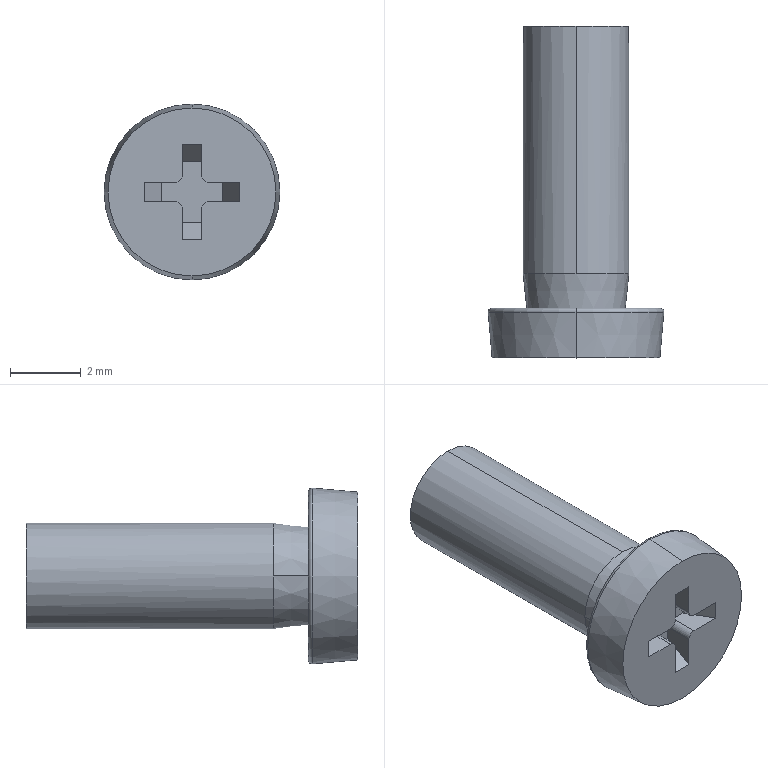Component | SolidWorks | cross recessed cheese head screws type a gb-1 | 1 solid | 28 faces | box 4.98 x 9.4 x 4.98 mm | volume 80 mm3 | plane 16 | cylinder 6 | cone 4 | torus 2 | commonest cylinder face diameters 0.4 x4 3 x2
STEP:
#1=COLOUR_RGB('',0.7922,0.8196,0.9333);
#2=FILL_AREA_STYLE_COLOUR('',#1);
#3=FILL_AREA_STYLE('',(#2));
#4=SURFACE_STYLE_FILL_AREA(#3);
#5=SURFACE_SIDE_STYLE('',(#4));
#6=SURFACE_STYLE_USAGE(.BOTH.,#5);
#7=PRESENTATION_STYLE_ASSIGNMENT((#6));
#8=CARTESIAN_POINT('',(0.2915,-2.334,0.9644));
#9=VERTEX_POINT('',#8);
#10=CARTESIAN_POINT('',(0.2915,-2.334,0.7683));
#11=VERTEX_POINT('',#10);
#12=CARTESIAN_POINT('',(0.2915,-2.334,0.8663));
#13=DIRECTION('',(0.,-1.,0.));
#14=DIRECTION('',(0.,0.,1.));
#15=AXIS2_PLACEMENT_3D('',#12,#13,#14);
#16=CIRCLE('',#15,0.09805);
#17=EDGE_CURVE('',#9,#11,#16,.T.);
#18=ORIENTED_EDGE('',*,*,#17,.F.);
#19=CARTESIAN_POINT('',(0.2915,-2.33,0.9604));
#20=VERTEX_POINT('',#19);
#21=CARTESIAN_POINT('',(0.2915,-2.334,0.9604));
#22=DIRECTION('',(-1.,0.,-0.));
#23=DIRECTION('',(0.,0.,1.));
#24=AXIS2_PLACEMENT_3D('',#21,#22,#23);
#25=CIRCLE('',#24,0.003937);
#26=EDGE_CURVE('',#9,#20,#25,.T.);
#27=ORIENTED_EDGE('',*,*,#26,.T.);
#28=CARTESIAN_POINT('',(0.2915,-2.33,0.7722));
#29=VERTEX_POINT('',#28);
#30=CARTESIAN_POINT('',(0.2915,-2.33,0.8663));
#31=DIRECTION('',(0.,1.,0.));
#32=DIRECTION('',(0.,0.,-1.));
#33=AXIS2_PLACEMENT_3D('',#30,#31,#32);
#34=CIRCLE('',#33,0.09413);
#35=EDGE_CURVE('',#29,#20,#34,.T.);
#36=ORIENTED_EDGE('',*,*,#35,.F.);
#37=CARTESIAN_POINT('',(0.2915,-2.334,0.7722));
#38=DIRECTION('',(1.,0.,0.));
#39=DIRECTION('',(0.,0.,-1.));
#40=AXIS2_PLACEMENT_3D('',#37,#38,#39);
#41=CIRCLE('',#40,0.003937);
#42=EDGE_CURVE('',#11,#29,#41,.T.);
#43=ORIENTED_EDGE('',*,*,#42,.F.);
#44=EDGE_LOOP('',(#18,#27,#36,#43));
#45=FACE_OUTER_BOUND('',#44,.T.);
#46=CARTESIAN_POINT('',(0.2915,-2.334,0.8663));
#47=DIRECTION('',(0.,1.,0.));
#48=DIRECTION('',(0.,0.,-1.));
#49=AXIS2_PLACEMENT_3D('',#46,#47,#48);
#50=TOROIDAL_SURFACE('',#49,0.09413,0.003937);
#51=ADVANCED_FACE('',(#45),#50,.T.);
#52=CARTESIAN_POINT('',(0.2915,-2.015,0.8072));
#53=VERTEX_POINT('',#52);
#54=CARTESIAN_POINT('',(0.2915,-2.015,0.9254));
#55=VERTEX_POINT('',#54);
#56=CARTESIAN_POINT('',(0.2915,-2.015,0.8663));
#57=DIRECTION('',(0.,1.,0.));
#58=DIRECTION('',(0.,0.,-1.));
#59=AXIS2_PLACEMENT_3D('',#56,#57,#58);
#60=CIRCLE('',#59,0.05906);
#61=EDGE_CURVE('',#53,#55,#60,.T.);
#62=ORIENTED_EDGE('',*,*,#61,.F.);
#63=CARTESIAN_POINT('',(0.2915,-2.291,0.8072));
#64=VERTEX_POINT('',#63);
#65=CARTESIAN_POINT('',(0.2915,-2.015,0.8072));
#66=DIRECTION('',(0.,-1.,0.));
#67=VECTOR('',#66,39.37);
#68=LINE('',#65,#67);
#69=EDGE_CURVE('',#53,#64,#68,.T.);
#70=ORIENTED_EDGE('',*,*,#69,.T.);
#71=CARTESIAN_POINT('',(0.2325,-2.291,0.8663));
#72=VERTEX_POINT('',#71);
#73=CARTESIAN_POINT('',(0.2915,-2.291,0.8663));
#74=DIRECTION('',(0.,1.,0.));
#75=DIRECTION('',(0.,0.,-1.));
#76=AXIS2_PLACEMENT_3D('',#73,#74,#75);
#77=CIRCLE('',#76,0.05906);
#78=EDGE_CURVE('',#64,#72,#77,.T.);
#79=ORIENTED_EDGE('',*,*,#78,.T.);
#80=CARTESIAN_POINT('',(0.2915,-2.291,0.9254));
#81=VERTEX_POINT('',#80);
#82=CARTESIAN_POINT('',(0.2915,-2.291,0.8663));
#83=DIRECTION('',(0.,1.,0.));
#84=DIRECTION('',(0.,0.,-1.));
#85=AXIS2_PLACEMENT_3D('',#82,#83,#84);
#86=CIRCLE('',#85,0.05906);
#87=EDGE_CURVE('',#72,#81,#86,.T.);
#88=ORIENTED_EDGE('',*,*,#87,.T.);
#89=CARTESIAN_POINT('',(0.2915,-2.015,0.9254));
#90=DIRECTION('',(0.,-1.,0.));
#91=VECTOR('',#90,39.37);
#92=LINE('',#89,#91);
#93=EDGE_CURVE('',#55,#81,#92,.T.);
#94=ORIENTED_EDGE('',*,*,#93,.F.);
#95=EDGE_LOOP('',(#62,#70,#79,#88,#94));
#96=FACE_OUTER_BOUND('',#95,.T.);
#97=CARTESIAN_POINT('',(0.2915,-2.015,0.8663));
#98=DIRECTION('',(0.,-1.,0.));
#99=DIRECTION('',(0.,0.,1.));
#100=AXIS2_PLACEMENT_3D('',#97,#98,#99);
#101=CYLINDRICAL_SURFACE('',#100,0.05906);
#102=ADVANCED_FACE('',(#96),#101,.T.);
#103=CARTESIAN_POINT('',(0.2915,-2.385,0.7727));
#104=VERTEX_POINT('',#103);
#105=CARTESIAN_POINT('',(0.2915,-2.385,0.9599));
#106=VERTEX_POINT('',#105);
#107=CARTESIAN_POINT('',(0.2915,-2.385,0.8663));
#108=DIRECTION('',(0.,1.,0.));
#109=DIRECTION('',(0.,0.,-1.));
#110=AXIS2_PLACEMENT_3D('',#107,#108,#109);
#111=CIRCLE('',#110,0.0936);
#112=EDGE_CURVE('',#104,#106,#111,.T.);
#113=ORIENTED_EDGE('',*,*,#112,.T.);
#114=CARTESIAN_POINT('',(0.2915,-2.33,0.9647));
#115=DIRECTION('',(-0.,0.9962,0.08716));
#116=VECTOR('',#115,39.37);
#117=LINE('',#114,#116);
#118=EDGE_CURVE('',#106,#9,#117,.T.);
#119=ORIENTED_EDGE('',*,*,#118,.T.);
#120=ORIENTED_EDGE('',*,*,#17,.T.);
#121=CARTESIAN_POINT('',(0.2915,-2.33,0.7679));
#122=DIRECTION('',(0.,0.9962,-0.08716));
#123=VECTOR('',#122,39.37);
#124=LINE('',#121,#123);
#125=EDGE_CURVE('',#104,#11,#124,.T.);
#126=ORIENTED_EDGE('',*,*,#125,.F.);
#127=EDGE_LOOP('',(#113,#119,#120,#126));
#128=FACE_OUTER_BOUND('',#127,.T.);
#129=CARTESIAN_POINT('',(0.2915,-2.33,0.8663));
#130=DIRECTION('',(0.,1.,0.));
#131=DIRECTION('',(0.,0.,-1.));
#132=AXIS2_PLACEMENT_3D('',#129,#130,#131);
#133=CONICAL_SURFACE('',#132,0.09843,0.08727);
#134=ADVANCED_FACE('',(#128),#133,.T.);
#135=CARTESIAN_POINT('',(0.2366,-2.33,0.8663));
#136=VERTEX_POINT('',#135);
#137=CARTESIAN_POINT('',(0.3464,-2.33,0.8663));
#138=VERTEX_POINT('',#137);
#139=CARTESIAN_POINT('',(0.2915,-2.33,0.8663));
#140=DIRECTION('',(0.,1.,0.));
#141=DIRECTION('',(0.,0.,-1.));
#142=AXIS2_PLACEMENT_3D('',#139,#140,#141);
#143=CIRCLE('',#142,0.05492);
#144=EDGE_CURVE('',#136,#138,#143,.T.);
#145=ORIENTED_EDGE('',*,*,#144,.T.);
#146=CARTESIAN_POINT('',(0.3506,-2.291,0.8663));
#147=VERTEX_POINT('',#146);
#148=CARTESIAN_POINT('',(0.3506,-2.291,0.8663));
#149=DIRECTION('',(0.1045,0.9945,0.));
#150=VECTOR('',#149,39.37);
#151=LINE('',#148,#150);
#152=EDGE_CURVE('',#138,#147,#151,.T.);
#153=ORIENTED_EDGE('',*,*,#152,.T.);
#154=CARTESIAN_POINT('',(0.2915,-2.291,0.8663));
#155=DIRECTION('',(0.,1.,0.));
#156=DIRECTION('',(0.,0.,-1.));
#157=AXIS2_PLACEMENT_3D('',#154,#155,#156);
#158=CIRCLE('',#157,0.05906);
#159=EDGE_CURVE('',#81,#147,#158,.T.);
#160=ORIENTED_EDGE('',*,*,#159,.F.);
#161=ORIENTED_EDGE('',*,*,#87,.F.);
#162=CARTESIAN_POINT('',(0.2325,-2.291,0.8663));
#163=DIRECTION('',(-0.1045,0.9945,0.));
#164=VECTOR('',#163,39.37);
#165=LINE('',#162,#164);
#166=EDGE_CURVE('',#136,#72,#165,.T.);
#167=ORIENTED_EDGE('',*,*,#166,.F.);
#168=EDGE_LOOP('',(#145,#153,#160,#161,#167));
#169=FACE_OUTER_BOUND('',#168,.T.);
#170=CARTESIAN_POINT('',(0.2915,-2.291,0.8663));
#171=DIRECTION('',(0.,1.,0.));
#172=DIRECTION('',(-1.,0.,0.));
#173=AXIS2_PLACEMENT_3D('',#170,#171,#172);
#174=CONICAL_SURFACE('',#173,0.05906,0.1047);
#175=ADVANCED_FACE('',(#169),#174,.T.);
#176=ORIENTED_EDGE('',*,*,#112,.F.);
#177=CARTESIAN_POINT('',(0.2915,-2.385,0.8663));
#178=DIRECTION('',(0.,1.,0.));
#179=DIRECTION('',(0.,0.,-1.));
#180=AXIS2_PLACEMENT_3D('',#177,#178,#179);
#181=CIRCLE('',#180,0.0936);
#182=EDGE_CURVE('',#106,#104,#181,.T.);
#183=ORIENTED_EDGE('',*,*,#182,.F.);
#184=EDGE_LOOP('',(#176,#183));
#185=FACE_OUTER_BOUND('',#184,.T.);
#186=CARTESIAN_POINT('',(0.2809,-2.385,0.8132));
#187=VERTEX_POINT('',#186);
#188=CARTESIAN_POINT('',(0.2809,-2.385,0.8478));
#189=VERTEX_POINT('',#188);
#190=CARTESIAN_POINT('',(0.2809,-2.385,0.8557));
#191=DIRECTION('',(-0.,0.,1.));
#192=VECTOR('',#191,39.37);
#193=LINE('',#190,#192);
#194=EDGE_CURVE('',#187,#189,#193,.T.);
#195=ORIENTED_EDGE('',*,*,#194,.T.);
#196=CARTESIAN_POINT('',(0.273,-2.385,0.8557));
#197=VERTEX_POINT('',#196);
#198=CARTESIAN_POINT('',(0.273,-2.385,0.8478));
#199=DIRECTION('',(0.,-1.,0.));
#200=DIRECTION('',(0.,0.,-1.));
#201=AXIS2_PLACEMENT_3D('',#198,#199,#200);
#202=CIRCLE('',#201,0.007874);
#203=EDGE_CURVE('',#189,#197,#202,.T.);
#204=ORIENTED_EDGE('',*,*,#203,.T.);
#205=CARTESIAN_POINT('',(0.2384,-2.385,0.8557));
#206=VERTEX_POINT('',#205);
#207=CARTESIAN_POINT('',(0.2384,-2.385,0.8557));
#208=DIRECTION('',(-1.,0.,0.));
#209=VECTOR('',#208,39.37);
#210=LINE('',#207,#209);
#211=EDGE_CURVE('',#197,#206,#210,.T.);
#212=ORIENTED_EDGE('',*,*,#211,.T.);
#213=CARTESIAN_POINT('',(0.2384,-2.385,0.8769));
#214=VERTEX_POINT('',#213);
#215=CARTESIAN_POINT('',(0.2384,-2.385,0.8769));
#216=DIRECTION('',(0.,0.,1.));
#217=VECTOR('',#216,39.37);
#218=LINE('',#215,#217);
#219=EDGE_CURVE('',#206,#214,#218,.T.);
#220=ORIENTED_EDGE('',*,*,#219,.T.);
#221=CARTESIAN_POINT('',(0.273,-2.385,0.8769));
#222=VERTEX_POINT('',#221);
#223=CARTESIAN_POINT('',(0.2384,-2.385,0.8769));
#224=DIRECTION('',(1.,0.,0.));
#225=VECTOR('',#224,39.37);
#226=LINE('',#223,#225);
#227=EDGE_CURVE('',#214,#222,#226,.T.);
#228=ORIENTED_EDGE('',*,*,#227,.T.);
#229=CARTESIAN_POINT('',(0.2809,-2.385,0.8848));
#230=VERTEX_POINT('',#229);
#231=CARTESIAN_POINT('',(0.273,-2.385,0.8848));
#232=DIRECTION('',(0.,-1.,0.));
#233=DIRECTION('',(0.,0.,-1.));
#234=AXIS2_PLACEMENT_3D('',#231,#232,#233);
#235=CIRCLE('',#234,0.007874);
#236=EDGE_CURVE('',#222,#230,#235,.T.);
#237=ORIENTED_EDGE('',*,*,#236,.T.);
#238=CARTESIAN_POINT('',(0.2809,-2.385,0.9195));
#239=VERTEX_POINT('',#238);
#240=CARTESIAN_POINT('',(0.2809,-2.385,0.9195));
#241=DIRECTION('',(0.,0.,1.));
#242=VECTOR('',#241,39.37);
#243=LINE('',#240,#242);
#244=EDGE_CURVE('',#230,#239,#243,.T.);
#245=ORIENTED_EDGE('',*,*,#244,.T.);
#246=CARTESIAN_POINT('',(0.3021,-2.385,0.9195));
#247=VERTEX_POINT('',#246);
#248=CARTESIAN_POINT('',(0.2809,-2.385,0.9195));
#249=DIRECTION('',(1.,0.,0.));
#250=VECTOR('',#249,39.37);
#251=LINE('',#248,#250);
#252=EDGE_CURVE('',#239,#247,#251,.T.);
#253=ORIENTED_EDGE('',*,*,#252,.T.);
#254=CARTESIAN_POINT('',(0.3021,-2.385,0.8848));
#255=VERTEX_POINT('',#254);
#256=CARTESIAN_POINT('',(0.3021,-2.385,0.9195));
#257=DIRECTION('',(0.,0.,-1.));
#258=VECTOR('',#257,39.37);
#259=LINE('',#256,#258);
#260=EDGE_CURVE('',#247,#255,#259,.T.);
#261=ORIENTED_EDGE('',*,*,#260,.T.);
#262=CARTESIAN_POINT('',(0.31,-2.385,0.8769));
#263=VERTEX_POINT('',#262);
#264=CARTESIAN_POINT('',(0.31,-2.385,0.8848));
#265=DIRECTION('',(0.,-1.,0.));
#266=DIRECTION('',(0.,0.,-1.));
#267=AXIS2_PLACEMENT_3D('',#264,#265,#266);
#268=CIRCLE('',#267,0.007874);
#269=EDGE_CURVE('',#255,#263,#268,.T.);
#270=ORIENTED_EDGE('',*,*,#269,.T.);
#271=CARTESIAN_POINT('',(0.3447,-2.385,0.8769));
#272=VERTEX_POINT('',#271);
#273=CARTESIAN_POINT('',(0.3021,-2.385,0.8769));
#274=DIRECTION('',(1.,0.,-0.));
#275=VECTOR('',#274,39.37);
#276=LINE('',#273,#275);
#277=EDGE_CURVE('',#263,#272,#276,.T.);
#278=ORIENTED_EDGE('',*,*,#277,.T.);
#279=CARTESIAN_POINT('',(0.3447,-2.385,0.8557));
#280=VERTEX_POINT('',#279);
#281=CARTESIAN_POINT('',(0.3447,-2.385,0.8769));
#282=DIRECTION('',(0.,0.,-1.));
#283=VECTOR('',#282,39.37);
#284=LINE('',#281,#283);
#285=EDGE_CURVE('',#272,#280,#284,.T.);
#286=ORIENTED_EDGE('',*,*,#285,.T.);
#287=CARTESIAN_POINT('',(0.31,-2.385,0.8557));
#288=VERTEX_POINT('',#287);
#289=CARTESIAN_POINT('',(0.3021,-2.385,0.8557));
#290=DIRECTION('',(-1.,0.,0.));
#291=VECTOR('',#290,39.37);
#292=LINE('',#289,#291);
#293=EDGE_CURVE('',#280,#288,#292,.T.);
#294=ORIENTED_EDGE('',*,*,#293,.T.);
#295=CARTESIAN_POINT('',(0.3021,-2.385,0.8478));
#296=VERTEX_POINT('',#295);
#297=CARTESIAN_POINT('',(0.31,-2.385,0.8478));
#298=DIRECTION('',(0.,-1.,0.));
#299=DIRECTION('',(0.,0.,-1.));
#300=AXIS2_PLACEMENT_3D('',#297,#298,#299);
#301=CIRCLE('',#300,0.007874);
#302=EDGE_CURVE('',#288,#296,#301,.T.);
#303=ORIENTED_EDGE('',*,*,#302,.T.);
#304=CARTESIAN_POINT('',(0.3021,-2.385,0.8132));
#305=VERTEX_POINT('',#304);
#306=CARTESIAN_POINT('',(0.3021,-2.385,0.8557));
#307=DIRECTION('',(-0.,0.,-1.));
#308=VECTOR('',#307,39.37);
#309=LINE('',#306,#308);
#310=EDGE_CURVE('',#296,#305,#309,.T.);
#311=ORIENTED_EDGE('',*,*,#310,.T.);
#312=CARTESIAN_POINT('',(0.2809,-2.385,0.8132));
#313=DIRECTION('',(-1.,0.,0.));
#314=VECTOR('',#313,39.37);
#315=LINE('',#312,#314);
#316=EDGE_CURVE('',#305,#187,#315,.T.);
#317=ORIENTED_EDGE('',*,*,#316,.T.);
#318=EDGE_LOOP('',(#195,#204,#212,#220,#228,#237,#245,#253,#261,#270,#278,#286,#294,#303,#311,#317));
#319=FACE_BOUND('',#318,.T.);
#320=CARTESIAN_POINT('',(0.2915,-2.385,0.8663));
#321=DIRECTION('',(0.,1.,0.));
#322=DIRECTION('',(0.,0.,-1.));
#323=AXIS2_PLACEMENT_3D('',#320,#321,#322);
#324=PLANE('',#323);
#325=ADVANCED_FACE('',(#185,#319),#324,.F.);
#326=ORIENTED_EDGE('',*,*,#152,.F.);
#327=CARTESIAN_POINT('',(0.2915,-2.33,0.8663));
#328=DIRECTION('',(0.,1.,0.));
#329=DIRECTION('',(0.,0.,-1.));
#330=AXIS2_PLACEMENT_3D('',#327,#328,#329);
#331=CIRCLE('',#330,0.05492);
#332=EDGE_CURVE('',#138,#136,#331,.T.);
#333=ORIENTED_EDGE('',*,*,#332,.T.);
#334=ORIENTED_EDGE('',*,*,#166,.T.);
#335=ORIENTED_EDGE('',*,*,#78,.F.);
#336=CARTESIAN_POINT('',(0.2915,-2.291,0.8663));
#337=DIRECTION('',(0.,1.,0.));
#338=DIRECTION('',(0.,0.,-1.));
#339=AXIS2_PLACEMENT_3D('',#336,#337,#338);
#340=CIRCLE('',#339,0.05906);
#341=EDGE_CURVE('',#147,#64,#340,.T.);
#342=ORIENTED_EDGE('',*,*,#341,.F.);
#343=EDGE_LOOP('',(#326,#333,#334,#335,#342));
#344=FACE_OUTER_BOUND('',#343,.T.);
#345=CARTESIAN_POINT('',(0.2915,-2.291,0.8663));
#346=DIRECTION('',(0.,1.,0.));
#347=DIRECTION('',(-1.,0.,0.));
#348=AXIS2_PLACEMENT_3D('',#345,#346,#347);
#349=CONICAL_SURFACE('',#348,0.05906,0.1047);
#350=ADVANCED_FACE('',(#344),#349,.T.);
#351=ORIENTED_EDGE('',*,*,#35,.T.);
#352=CARTESIAN_POINT('',(0.2915,-2.33,0.8663));
#353=DIRECTION('',(0.,1.,0.));
#354=DIRECTION('',(0.,0.,-1.));
#355=AXIS2_PLACEMENT_3D('',#352,#353,#354);
#356=CIRCLE('',#355,0.09413);
#357=EDGE_CURVE('',#20,#29,#356,.T.);
#358=ORIENTED_EDGE('',*,*,#357,.T.);
#359=EDGE_LOOP('',(#351,#358));
#360=FACE_OUTER_BOUND('',#359,.T.);
#361=ORIENTED_EDGE('',*,*,#144,.F.);
#362=ORIENTED_EDGE('',*,*,#332,.F.);
#363=EDGE_LOOP('',(#361,#362));
#364=FACE_BOUND('',#363,.T.);
#365=CARTESIAN_POINT('',(0.2915,-2.33,0.8663));
#366=DIRECTION('',(0.,1.,0.));
#367=DIRECTION('',(0.,0.,-1.));
#368=AXIS2_PLACEMENT_3D('',#365,#366,#367);
#369=PLANE('',#368);
#370=ADVANCED_FACE('',(#360,#364),#369,.T.);
#371=ORIENTED_EDGE('',*,*,#118,.F.);
#372=ORIENTED_EDGE('',*,*,#182,.T.);
#373=ORIENTED_EDGE('',*,*,#125,.T.);
#374=CARTESIAN_POINT('',(0.2915,-2.334,0.8663));
#375=DIRECTION('',(0.,-1.,0.));
#376=DIRECTION('',(0.,0.,1.));
#377=AXIS2_PLACEMENT_3D('',#374,#375,#376);
#378=CIRCLE('',#377,0.09805);
#379=EDGE_CURVE('',#11,#9,#378,.T.);
#380=ORIENTED_EDGE('',*,*,#379,.T.);
#381=EDGE_LOOP('',(#371,#372,#373,#380));
#382=FACE_OUTER_BOUND('',#381,.T.);
#383=CARTESIAN_POINT('',(0.2915,-2.33,0.8663));
#384=DIRECTION('',(0.,1.,0.));
#385=DIRECTION('',(0.,0.,-1.));
#386=AXIS2_PLACEMENT_3D('',#383,#384,#385);
#387=CONICAL_SURFACE('',#386,0.09843,0.08727);
#388=ADVANCED_FACE('',(#382),#387,.T.);
#389=ORIENTED_EDGE('',*,*,#69,.F.);
#390=CARTESIAN_POINT('',(0.2915,-2.015,0.8663));
#391=DIRECTION('',(0.,1.,0.));
#392=DIRECTION('',(0.,0.,-1.));
#393=AXIS2_PLACEMENT_3D('',#390,#391,#392);
#394=CIRCLE('',#393,0.05906);
#395=EDGE_CURVE('',#55,#53,#394,.T.);
#396=ORIENTED_EDGE('',*,*,#395,.F.);
#397=ORIENTED_EDGE('',*,*,#93,.T.);
#398=ORIENTED_EDGE('',*,*,#159,.T.);
#399=ORIENTED_EDGE('',*,*,#341,.T.);
#400=EDGE_LOOP('',(#389,#396,#397,#398,#399));
#401=FACE_OUTER_BOUND('',#400,.T.);
#402=CARTESIAN_POINT('',(0.2915,-2.015,0.8663));
#403=DIRECTION('',(0.,-1.,0.));
#404=DIRECTION('',(0.,0.,1.));
#405=AXIS2_PLACEMENT_3D('',#402,#403,#404);
#406=CYLINDRICAL_SURFACE('',#405,0.05906);
#407=ADVANCED_FACE('',(#401),#406,.T.);
#408=ORIENTED_EDGE('',*,*,#395,.T.);
#409=ORIENTED_EDGE('',*,*,#61,.T.);
#410=EDGE_LOOP('',(#408,#409));
#411=FACE_OUTER_BOUND('',#410,.T.);
#412=CARTESIAN_POINT('',(0.2915,-2.015,0.8663));
#413=DIRECTION('',(0.,1.,0.));
#414=DIRECTION('',(0.,0.,-1.));
#415=AXIS2_PLACEMENT_3D('',#412,#413,#414);
#416=PLANE('',#415);
#417=ADVANCED_FACE('',(#411),#416,.T.);
#418=CARTESIAN_POINT('',(0.2575,-2.352,0.8769));
#419=VERTEX_POINT('',#418);
#420=CARTESIAN_POINT('',(0.273,-2.352,0.8769));
#421=VERTEX_POINT('',#420);
#422=CARTESIAN_POINT('',(0.2384,-2.352,0.8769));
#423=DIRECTION('',(1.,0.,0.));
#424=VECTOR('',#423,39.37);
#425=LINE('',#422,#424);
#426=EDGE_CURVE('',#419,#421,#425,.T.);
#427=ORIENTED_EDGE('',*,*,#426,.T.);
#428=CARTESIAN_POINT('',(0.273,-2.352,0.8769));
#429=DIRECTION('',(0.,-1.,0.));
#430=VECTOR('',#429,39.37);
#431=LINE('',#428,#430);
#432=EDGE_CURVE('',#421,#222,#431,.T.);
#433=ORIENTED_EDGE('',*,*,#432,.T.);
#434=ORIENTED_EDGE('',*,*,#227,.F.);
#435=CARTESIAN_POINT('',(0.2527,-2.36,0.8769));
#436=DIRECTION('',(-0.5,-0.866,-0.));
#437=VECTOR('',#436,39.37);
#438=LINE('',#435,#437);
#439=EDGE_CURVE('',#419,#214,#438,.T.);
#440=ORIENTED_EDGE('',*,*,#439,.F.);
#441=EDGE_LOOP('',(#427,#433,#434,#440));
#442=FACE_OUTER_BOUND('',#441,.T.);
#443=CARTESIAN_POINT('',(0.2384,-2.352,0.8769));
#444=DIRECTION('',(0.,0.,-1.));
#445=DIRECTION('',(-1.,0.,-0.));
#446=AXIS2_PLACEMENT_3D('',#443,#444,#445);
#447=PLANE('',#446);
#448=ADVANCED_FACE('',(#442),#447,.T.);
#449=ORIENTED_EDGE('',*,*,#244,.F.);
#450=CARTESIAN_POINT('',(0.2809,-2.352,0.8848));
#451=VERTEX_POINT('',#450);
#452=CARTESIAN_POINT('',(0.2809,-2.352,0.8848));
#453=DIRECTION('',(0.,1.,0.));
#454=VECTOR('',#453,39.37);
#455=LINE('',#452,#454);
#456=EDGE_CURVE('',#230,#451,#455,.T.);
#457=ORIENTED_EDGE('',*,*,#456,.T.);
#458=CARTESIAN_POINT('',(0.2809,-2.352,0.9004));
#459=VERTEX_POINT('',#458);
#460=CARTESIAN_POINT('',(0.2809,-2.352,0.9195));
#461=DIRECTION('',(0.,0.,1.));
#462=VECTOR('',#461,39.37);
#463=LINE('',#460,#462);
#464=EDGE_CURVE('',#451,#459,#463,.T.);
#465=ORIENTED_EDGE('',*,*,#464,.T.);
#466=CARTESIAN_POINT('',(0.2809,-2.385,0.9195));
#467=DIRECTION('',(0.,-0.866,0.5));
#468=VECTOR('',#467,39.37);
#469=LINE('',#466,#468);
#470=EDGE_CURVE('',#459,#239,#469,.T.);
#471=ORIENTED_EDGE('',*,*,#470,.T.);
#472=EDGE_LOOP('',(#449,#457,#465,#471));
#473=FACE_OUTER_BOUND('',#472,.T.);
#474=CARTESIAN_POINT('',(0.2809,-2.352,0.9195));
#475=DIRECTION('',(1.,0.,-0.));
#476=DIRECTION('',(-0.,0.,-1.));
#477=AXIS2_PLACEMENT_3D('',#474,#475,#476);
#478=PLANE('',#477);
#479=ADVANCED_FACE('',(#473),#478,.T.);
#480=ORIENTED_EDGE('',*,*,#252,.F.);
#481=ORIENTED_EDGE('',*,*,#470,.F.);
#482=CARTESIAN_POINT('',(0.3021,-2.352,0.9004));
#483=VERTEX_POINT('',#482);
#484=CARTESIAN_POINT('',(0.2809,-2.352,0.9004));
#485=DIRECTION('',(1.,0.,0.));
#486=VECTOR('',#485,39.37);
#487=LINE('',#484,#486);
#488=EDGE_CURVE('',#459,#483,#487,.T.);
#489=ORIENTED_EDGE('',*,*,#488,.T.);
#490=CARTESIAN_POINT('',(0.3021,-2.36,0.9051));
#491=DIRECTION('',(-0.,-0.866,0.5));
#492=VECTOR('',#491,39.37);
#493=LINE('',#490,#492);
#494=EDGE_CURVE('',#483,#247,#493,.T.);
#495=ORIENTED_EDGE('',*,*,#494,.T.);
#496=EDGE_LOOP('',(#480,#481,#489,#495));
#497=FACE_OUTER_BOUND('',#496,.T.);
#498=CARTESIAN_POINT('',(0.2809,-2.385,0.9195));
#499=DIRECTION('',(0.,-0.5,-0.866));
#500=DIRECTION('',(0.,-0.866,0.5));
#501=AXIS2_PLACEMENT_3D('',#498,#499,#500);
#502=PLANE('',#501);
#503=ADVANCED_FACE('',(#497),#502,.T.);
#504=CARTESIAN_POINT('',(0.3021,-2.352,0.8848));
#505=VERTEX_POINT('',#504);
#506=CARTESIAN_POINT('',(0.3021,-2.352,0.9195));
#507=DIRECTION('',(0.,0.,-1.));
#508=VECTOR('',#507,39.37);
#509=LINE('',#506,#508);
#510=EDGE_CURVE('',#483,#505,#509,.T.);
#511=ORIENTED_EDGE('',*,*,#510,.T.);
#512=CARTESIAN_POINT('',(0.3021,-2.352,0.8848));
#513=DIRECTION('',(0.,-1.,0.));
#514=VECTOR('',#513,39.37);
#515=LINE('',#512,#514);
#516=EDGE_CURVE('',#505,#255,#515,.T.);
#517=ORIENTED_EDGE('',*,*,#516,.T.);
#518=ORIENTED_EDGE('',*,*,#260,.F.);
#519=ORIENTED_EDGE('',*,*,#494,.F.);
#520=EDGE_LOOP('',(#511,#517,#518,#519));
#521=FACE_OUTER_BOUND('',#520,.T.);
#522=CARTESIAN_POINT('',(0.3021,-2.352,0.9195));
#523=DIRECTION('',(-1.,0.,-0.));
#524=DIRECTION('',(-0.,0.,1.));
#525=AXIS2_PLACEMENT_3D('',#522,#523,#524);
#526=PLANE('',#525);
#527=ADVANCED_FACE('',(#521),#526,.T.);
#528=ORIENTED_EDGE('',*,*,#277,.F.);
#529=CARTESIAN_POINT('',(0.31,-2.352,0.8769));
#530=VERTEX_POINT('',#529);
#531=CARTESIAN_POINT('',(0.31,-2.352,0.8769));
#532=DIRECTION('',(0.,1.,0.));
#533=VECTOR('',#532,39.37);
#534=LINE('',#531,#533);
#535=EDGE_CURVE('',#263,#530,#534,.T.);
#536=ORIENTED_EDGE('',*,*,#535,.T.);
#537=CARTESIAN_POINT('',(0.3256,-2.352,0.8769));
#538=VERTEX_POINT('',#537);
#539=CARTESIAN_POINT('',(0.3021,-2.352,0.8769));
#540=DIRECTION('',(1.,0.,-0.));
#541=VECTOR('',#540,39.37);
#542=LINE('',#539,#541);
#543=EDGE_CURVE('',#530,#538,#542,.T.);
#544=ORIENTED_EDGE('',*,*,#543,.T.);
#545=CARTESIAN_POINT('',(0.3447,-2.385,0.8769));
#546=DIRECTION('',(0.5,-0.866,-0.));
#547=VECTOR('',#546,39.37);
#548=LINE('',#545,#547);
#549=EDGE_CURVE('',#538,#272,#548,.T.);
#550=ORIENTED_EDGE('',*,*,#549,.T.);
#551=EDGE_LOOP('',(#528,#536,#544,#550));
#552=FACE_OUTER_BOUND('',#551,.T.);
#553=CARTESIAN_POINT('',(0.3021,-2.352,0.8769));
#554=DIRECTION('',(-0.,0.,-1.));
#555=DIRECTION('',(-1.,0.,0.));
#556=AXIS2_PLACEMENT_3D('',#553,#554,#555);
#557=PLANE('',#556);
#558=ADVANCED_FACE('',(#552),#557,.T.);
#559=ORIENTED_EDGE('',*,*,#285,.F.);
#560=ORIENTED_EDGE('',*,*,#549,.F.);
#561=CARTESIAN_POINT('',(0.3256,-2.352,0.8557));
#562=VERTEX_POINT('',#561);
#563=CARTESIAN_POINT('',(0.3256,-2.352,0.8769));
#564=DIRECTION('',(0.,0.,-1.));
#565=VECTOR('',#564,39.37);
#566=LINE('',#563,#565);
#567=EDGE_CURVE('',#538,#562,#566,.T.);
#568=ORIENTED_EDGE('',*,*,#567,.T.);
#569=CARTESIAN_POINT('',(0.3197,-2.342,0.8557));
#570=DIRECTION('',(0.5,-0.866,-0.));
#571=VECTOR('',#570,39.37);
#572=LINE('',#569,#571);
#573=EDGE_CURVE('',#562,#280,#572,.T.);
#574=ORIENTED_EDGE('',*,*,#573,.T.);
#575=EDGE_LOOP('',(#559,#560,#568,#574));
#576=FACE_OUTER_BOUND('',#575,.T.);
#577=CARTESIAN_POINT('',(0.3447,-2.385,0.8769));
#578=DIRECTION('',(-0.866,-0.5,0.));
#579=DIRECTION('',(0.5,-0.866,0.));
#580=AXIS2_PLACEMENT_3D('',#577,#578,#579);
#581=PLANE('',#580);
#582=ADVANCED_FACE('',(#576),#581,.T.);
#583=CARTESIAN_POINT('',(0.31,-2.352,0.8557));
#584=VERTEX_POINT('',#583);
#585=CARTESIAN_POINT('',(0.3021,-2.352,0.8557));
#586=DIRECTION('',(-1.,0.,0.));
#587=VECTOR('',#586,39.37);
#588=LINE('',#585,#587);
#589=EDGE_CURVE('',#562,#584,#588,.T.);
#590=ORIENTED_EDGE('',*,*,#589,.T.);
#591=CARTESIAN_POINT('',(0.31,-2.352,0.8557));
#592=DIRECTION('',(0.,-1.,0.));
#593=VECTOR('',#592,39.37);
#594=LINE('',#591,#593);
#595=EDGE_CURVE('',#584,#288,#594,.T.);
#596=ORIENTED_EDGE('',*,*,#595,.T.);
#597=ORIENTED_EDGE('',*,*,#293,.F.);
#598=ORIENTED_EDGE('',*,*,#573,.F.);
#599=EDGE_LOOP('',(#590,#596,#597,#598));
#600=FACE_OUTER_BOUND('',#599,.T.);
#601=CARTESIAN_POINT('',(0.3021,-2.352,0.8557));
#602=DIRECTION('',(0.,0.,1.));
#603=DIRECTION('',(1.,0.,-0.));
#604=AXIS2_PLACEMENT_3D('',#601,#602,#603);
#605=PLANE('',#604);
#606=ADVANCED_FACE('',(#600),#605,.T.);
#607=ORIENTED_EDGE('',*,*,#310,.F.);
#608=CARTESIAN_POINT('',(0.3021,-2.352,0.8478));
#609=VERTEX_POINT('',#608);
#610=CARTESIAN_POINT('',(0.3021,-2.352,0.8478));
#611=DIRECTION('',(0.,1.,0.));
#612=VECTOR('',#611,39.37);
#613=LINE('',#610,#612);
#614=EDGE_CURVE('',#296,#609,#613,.T.);
#615=ORIENTED_EDGE('',*,*,#614,.T.);
#616=CARTESIAN_POINT('',(0.3021,-2.352,0.8322));
#617=VERTEX_POINT('',#616);
#618=CARTESIAN_POINT('',(0.3021,-2.352,0.8557));
#619=DIRECTION('',(-0.,0.,-1.));
#620=VECTOR('',#619,39.37);
#621=LINE('',#618,#620);
#622=EDGE_CURVE('',#609,#617,#621,.T.);
#623=ORIENTED_EDGE('',*,*,#622,.T.);
#624=CARTESIAN_POINT('',(0.3021,-2.385,0.8132));
#625=DIRECTION('',(-0.,-0.866,-0.5));
#626=VECTOR('',#625,39.37);
#627=LINE('',#624,#626);
#628=EDGE_CURVE('',#617,#305,#627,.T.);
#629=ORIENTED_EDGE('',*,*,#628,.T.);
#630=EDGE_LOOP('',(#607,#615,#623,#629));
#631=FACE_OUTER_BOUND('',#630,.T.);
#632=CARTESIAN_POINT('',(0.3021,-2.352,0.8557));
#633=DIRECTION('',(-1.,0.,0.));
#634=DIRECTION('',(0.,0.,1.));
#635=AXIS2_PLACEMENT_3D('',#632,#633,#634);
#636=PLANE('',#635);
#637=ADVANCED_FACE('',(#631),#636,.T.);
#638=ORIENTED_EDGE('',*,*,#316,.F.);
#639=ORIENTED_EDGE('',*,*,#628,.F.);
#640=CARTESIAN_POINT('',(0.2809,-2.352,0.8322));
#641=VERTEX_POINT('',#640);
#642=CARTESIAN_POINT('',(0.2809,-2.352,0.8322));
#643=DIRECTION('',(-1.,0.,0.));
#644=VECTOR('',#643,39.37);
#645=LINE('',#642,#644);
#646=EDGE_CURVE('',#617,#641,#645,.T.);
#647=ORIENTED_EDGE('',*,*,#646,.T.);
#648=CARTESIAN_POINT('',(0.2809,-2.342,0.8381));
#649=DIRECTION('',(0.,-0.866,-0.5));
#650=VECTOR('',#649,39.37);
#651=LINE('',#648,#650);
#652=EDGE_CURVE('',#641,#187,#651,.T.);
#653=ORIENTED_EDGE('',*,*,#652,.T.);
#654=EDGE_LOOP('',(#638,#639,#647,#653));
#655=FACE_OUTER_BOUND('',#654,.T.);
#656=CARTESIAN_POINT('',(0.2809,-2.385,0.8132));
#657=DIRECTION('',(0.,-0.5,0.866));
#658=DIRECTION('',(0.,0.866,0.5));
#659=AXIS2_PLACEMENT_3D('',#656,#657,#658);
#660=PLANE('',#659);
#661=ADVANCED_FACE('',(#655),#660,.T.);
#662=CARTESIAN_POINT('',(0.2809,-2.352,0.8478));
#663=VERTEX_POINT('',#662);
#664=CARTESIAN_POINT('',(0.2809,-2.352,0.8557));
#665=DIRECTION('',(-0.,0.,1.));
#666=VECTOR('',#665,39.37);
#667=LINE('',#664,#666);
#668=EDGE_CURVE('',#641,#663,#667,.T.);
#669=ORIENTED_EDGE('',*,*,#668,.T.);
#670=CARTESIAN_POINT('',(0.2809,-2.352,0.8478));
#671=DIRECTION('',(0.,-1.,0.));
#672=VECTOR('',#671,39.37);
#673=LINE('',#670,#672);
#674=EDGE_CURVE('',#663,#189,#673,.T.);
#675=ORIENTED_EDGE('',*,*,#674,.T.);
#676=ORIENTED_EDGE('',*,*,#194,.F.);
#677=ORIENTED_EDGE('',*,*,#652,.F.);
#678=EDGE_LOOP('',(#669,#675,#676,#677));
#679=FACE_OUTER_BOUND('',#678,.T.);
#680=CARTESIAN_POINT('',(0.2809,-2.352,0.8557));
#681=DIRECTION('',(1.,0.,0.));
#682=DIRECTION('',(0.,0.,-1.));
#683=AXIS2_PLACEMENT_3D('',#680,#681,#682);
#684=PLANE('',#683);
#685=ADVANCED_FACE('',(#679),#684,.T.);
#686=ORIENTED_EDGE('',*,*,#211,.F.);
#687=CARTESIAN_POINT('',(0.273,-2.352,0.8557));
#688=VERTEX_POINT('',#687);
#689=CARTESIAN_POINT('',(0.273,-2.352,0.8557));
#690=DIRECTION('',(0.,1.,0.));
#691=VECTOR('',#690,39.37);
#692=LINE('',#689,#691);
#693=EDGE_CURVE('',#197,#688,#692,.T.);
#694=ORIENTED_EDGE('',*,*,#693,.T.);
#695=CARTESIAN_POINT('',(0.2575,-2.352,0.8557));
#696=VERTEX_POINT('',#695);
#697=CARTESIAN_POINT('',(0.2384,-2.352,0.8557));
#698=DIRECTION('',(-1.,0.,0.));
#699=VECTOR('',#698,39.37);
#700=LINE('',#697,#699);
#701=EDGE_CURVE('',#688,#696,#700,.T.);
#702=ORIENTED_EDGE('',*,*,#701,.T.);
#703=CARTESIAN_POINT('',(0.2384,-2.385,0.8557));
#704=DIRECTION('',(-0.5,-0.866,0.));
#705=VECTOR('',#704,39.37);
#706=LINE('',#703,#705);
#707=EDGE_CURVE('',#696,#206,#706,.T.);
#708=ORIENTED_EDGE('',*,*,#707,.T.);
#709=EDGE_LOOP('',(#686,#694,#702,#708));
#710=FACE_OUTER_BOUND('',#709,.T.);
#711=CARTESIAN_POINT('',(0.2384,-2.352,0.8557));
#712=DIRECTION('',(0.,0.,1.));
#713=DIRECTION('',(1.,0.,-0.));
#714=AXIS2_PLACEMENT_3D('',#711,#712,#713);
#715=PLANE('',#714);
#716=ADVANCED_FACE('',(#710),#715,.T.);
#717=ORIENTED_EDGE('',*,*,#219,.F.);
#718=ORIENTED_EDGE('',*,*,#707,.F.);
#719=CARTESIAN_POINT('',(0.2575,-2.352,0.8769));
#720=DIRECTION('',(0.,0.,1.));
#721=VECTOR('',#720,39.37);
#722=LINE('',#719,#721);
#723=EDGE_CURVE('',#696,#419,#722,.T.);
#724=ORIENTED_EDGE('',*,*,#723,.T.);
#725=ORIENTED_EDGE('',*,*,#439,.T.);
#726=EDGE_LOOP('',(#717,#718,#724,#725));
#727=FACE_OUTER_BOUND('',#726,.T.);
#728=CARTESIAN_POINT('',(0.2384,-2.385,0.8769));
#729=DIRECTION('',(0.866,-0.5,0.));
#730=DIRECTION('',(0.5,0.866,0.));
#731=AXIS2_PLACEMENT_3D('',#728,#729,#730);
#732=PLANE('',#731);
#733=ADVANCED_FACE('',(#727),#732,.T.);
#734=ORIENTED_EDGE('',*,*,#426,.F.);
#735=ORIENTED_EDGE('',*,*,#723,.F.);
#736=ORIENTED_EDGE('',*,*,#701,.F.);
#737=CARTESIAN_POINT('',(0.273,-2.352,0.8478));
#738=DIRECTION('',(0.,1.,0.));
#739=DIRECTION('',(0.,0.,-1.));
#740=AXIS2_PLACEMENT_3D('',#737,#738,#739);
#741=CIRCLE('',#740,0.007874);
#742=EDGE_CURVE('',#688,#663,#741,.T.);
#743=ORIENTED_EDGE('',*,*,#742,.T.);
#744=ORIENTED_EDGE('',*,*,#668,.F.);
#745=ORIENTED_EDGE('',*,*,#646,.F.);
#746=ORIENTED_EDGE('',*,*,#622,.F.);
#747=CARTESIAN_POINT('',(0.31,-2.352,0.8478));
#748=DIRECTION('',(0.,1.,0.));
#749=DIRECTION('',(0.,0.,-1.));
#750=AXIS2_PLACEMENT_3D('',#747,#748,#749);
#751=CIRCLE('',#750,0.007874);
#752=EDGE_CURVE('',#609,#584,#751,.T.);
#753=ORIENTED_EDGE('',*,*,#752,.T.);
#754=ORIENTED_EDGE('',*,*,#589,.F.);
#755=ORIENTED_EDGE('',*,*,#567,.F.);
#756=ORIENTED_EDGE('',*,*,#543,.F.);
#757=CARTESIAN_POINT('',(0.31,-2.352,0.8848));
#758=DIRECTION('',(0.,1.,0.));
#759=DIRECTION('',(0.,0.,-1.));
#760=AXIS2_PLACEMENT_3D('',#757,#758,#759);
#761=CIRCLE('',#760,0.007874);
#762=EDGE_CURVE('',#530,#505,#761,.T.);
#763=ORIENTED_EDGE('',*,*,#762,.T.);
#764=ORIENTED_EDGE('',*,*,#510,.F.);
#765=ORIENTED_EDGE('',*,*,#488,.F.);
#766=ORIENTED_EDGE('',*,*,#464,.F.);
#767=CARTESIAN_POINT('',(0.273,-2.352,0.8848));
#768=DIRECTION('',(0.,1.,0.));
#769=DIRECTION('',(0.,0.,-1.));
#770=AXIS2_PLACEMENT_3D('',#767,#768,#769);
#771=CIRCLE('',#770,0.007874);
#772=EDGE_CURVE('',#451,#421,#771,.T.);
#773=ORIENTED_EDGE('',*,*,#772,.T.);
#774=EDGE_LOOP('',(#734,#735,#736,#743,#744,#745,#746,#753,#754,#755,#756,#763,#764,#765,#766,#773));
#775=FACE_OUTER_BOUND('',#774,.T.);
#776=CARTESIAN_POINT('',(0.3021,-2.352,0.8769));
#777=DIRECTION('',(0.,1.,0.));
#778=DIRECTION('',(0.,0.,-1.));
#779=AXIS2_PLACEMENT_3D('',#776,#777,#778);
#780=PLANE('',#779);
#781=ADVANCED_FACE('',(#775),#780,.F.);
#782=ORIENTED_EDGE('',*,*,#742,.F.);
#783=ORIENTED_EDGE('',*,*,#693,.F.);
#784=ORIENTED_EDGE('',*,*,#203,.F.);
#785=ORIENTED_EDGE('',*,*,#674,.F.);
#786=EDGE_LOOP('',(#782,#783,#784,#785));
#787=FACE_OUTER_BOUND('',#786,.T.);
#788=CARTESIAN_POINT('',(0.273,-2.352,0.8478));
#789=DIRECTION('',(0.,-1.,0.));
#790=DIRECTION('',(0.,0.,1.));
#791=AXIS2_PLACEMENT_3D('',#788,#789,#790);
#792=CYLINDRICAL_SURFACE('',#791,0.007874);
#793=ADVANCED_FACE('',(#787),#792,.T.);
#794=ORIENTED_EDGE('',*,*,#772,.F.);
#795=ORIENTED_EDGE('',*,*,#456,.F.);
#796=ORIENTED_EDGE('',*,*,#236,.F.);
#797=ORIENTED_EDGE('',*,*,#432,.F.);
#798=EDGE_LOOP('',(#794,#795,#796,#797));
#799=FACE_OUTER_BOUND('',#798,.T.);
#800=CARTESIAN_POINT('',(0.273,-2.352,0.8848));
#801=DIRECTION('',(0.,-1.,0.));
#802=DIRECTION('',(0.,0.,1.));
#803=AXIS2_PLACEMENT_3D('',#800,#801,#802);
#804=CYLINDRICAL_SURFACE('',#803,0.007874);
#805=ADVANCED_FACE('',(#799),#804,.T.);
#806=ORIENTED_EDGE('',*,*,#752,.F.);
#807=ORIENTED_EDGE('',*,*,#614,.F.);
#808=ORIENTED_EDGE('',*,*,#302,.F.);
#809=ORIENTED_EDGE('',*,*,#595,.F.);
#810=EDGE_LOOP('',(#806,#807,#808,#809));
#811=FACE_OUTER_BOUND('',#810,.T.);
#812=CARTESIAN_POINT('',(0.31,-2.352,0.8478));
#813=DIRECTION('',(0.,-1.,0.));
#814=DIRECTION('',(0.,0.,1.));
#815=AXIS2_PLACEMENT_3D('',#812,#813,#814);
#816=CYLINDRICAL_SURFACE('',#815,0.007874);
#817=ADVANCED_FACE('',(#811),#816,.T.);
#818=ORIENTED_EDGE('',*,*,#762,.F.);
#819=ORIENTED_EDGE('',*,*,#535,.F.);
#820=ORIENTED_EDGE('',*,*,#269,.F.);
#821=ORIENTED_EDGE('',*,*,#516,.F.);
#822=EDGE_LOOP('',(#818,#819,#820,#821));
#823=FACE_OUTER_BOUND('',#822,.T.);
#824=CARTESIAN_POINT('',(0.31,-2.352,0.8848));
#825=DIRECTION('',(0.,-1.,0.));
#826=DIRECTION('',(0.,0.,1.));
#827=AXIS2_PLACEMENT_3D('',#824,#825,#826);
#828=CYLINDRICAL_SURFACE('',#827,0.007874);
#829=ADVANCED_FACE('',(#823),#828,.T.);
#830=ORIENTED_EDGE('',*,*,#26,.F.);
#831=ORIENTED_EDGE('',*,*,#379,.F.);
#832=ORIENTED_EDGE('',*,*,#42,.T.);
#833=ORIENTED_EDGE('',*,*,#357,.F.);
#834=EDGE_LOOP('',(#830,#831,#832,#833));
#835=FACE_OUTER_BOUND('',#834,.T.);
#836=CARTESIAN_POINT('',(0.2915,-2.334,0.8663));
#837=DIRECTION('',(0.,1.,0.));
#838=DIRECTION('',(0.,0.,-1.));
#839=AXIS2_PLACEMENT_3D('',#836,#837,#838);
#840=TOROIDAL_SURFACE('',#839,0.09413,0.003937);
#841=ADVANCED_FACE('',(#835),#840,.T.);
#842=CLOSED_SHELL('',(#51,#102,#134,#175,#325,#350,#370,#388,#407,#417,#448,#479,#503,#527,#558,#582,#606,#637,#661,#685,#716,#733,#781,#793,#805,#817,#829,#841));
#843=MANIFOLD_SOLID_BREP('',#842);
#844=STYLED_ITEM('',(#7),#843);
#845=(LENGTH_UNIT()NAMED_UNIT(*)SI_UNIT($,.METRE.));
#846=LENGTH_MEASURE_WITH_UNIT(LENGTH_MEASURE(0.0254),#845);
#847=DIMENSIONAL_EXPONENTS(1.,0.,0.,0.,0.,0.,0.);
#848=(CONVERSION_BASED_UNIT('',#846)LENGTH_UNIT()NAMED_UNIT(#847));
#849=UNCERTAINTY_MEASURE_WITH_UNIT(LENGTH_MEASURE(0.00001),#848,'','');
#850=(NAMED_UNIT(*)PLANE_ANGLE_UNIT()SI_UNIT($,.RADIAN.));
#851=(NAMED_UNIT(*)SI_UNIT($,.STERADIAN.)SOLID_ANGLE_UNIT());
#852=(GEOMETRIC_REPRESENTATION_CONTEXT(3)GLOBAL_UNCERTAINTY_ASSIGNED_CONTEXT((#849))GLOBAL_UNIT_ASSIGNED_CONTEXT((#848,#850,#851))REPRESENTATION_CONTEXT('',''));
#853=MECHANICAL_DESIGN_GEOMETRIC_PRESENTATION_REPRESENTATION('',(#844),#852);
#854=PRESENTATION_LAYER_ASSIGNMENT('','',(#844));
#855=CARTESIAN_POINT('',(0.,0.,0.));
#856=DIRECTION('',(0.,0.,1.));
#857=DIRECTION('',(1.,0.,0.));
#858=AXIS2_PLACEMENT_3D('',#855,#856,#857);
#859=(LENGTH_UNIT()NAMED_UNIT(*)SI_UNIT($,.METRE.));
#860=LENGTH_MEASURE_WITH_UNIT(LENGTH_MEASURE(0.0254),#859);
#861=DIMENSIONAL_EXPONENTS(1.,0.,0.,0.,0.,0.,0.);
#862=(CONVERSION_BASED_UNIT('',#860)LENGTH_UNIT()NAMED_UNIT(#861));
#863=UNCERTAINTY_MEASURE_WITH_UNIT(LENGTH_MEASURE(0.00001),#862,'','');
#864=(NAMED_UNIT(*)PLANE_ANGLE_UNIT()SI_UNIT($,.RADIAN.));
#865=(NAMED_UNIT(*)SI_UNIT($,.STERADIAN.)SOLID_ANGLE_UNIT());
#866=(GEOMETRIC_REPRESENTATION_CONTEXT(3)GLOBAL_UNCERTAINTY_ASSIGNED_CONTEXT((#863))GLOBAL_UNIT_ASSIGNED_CONTEXT((#862,#864,#865))REPRESENTATION_CONTEXT('',''));
#867=ADVANCED_BREP_SHAPE_REPRESENTATION('',(#843,#858),#866);